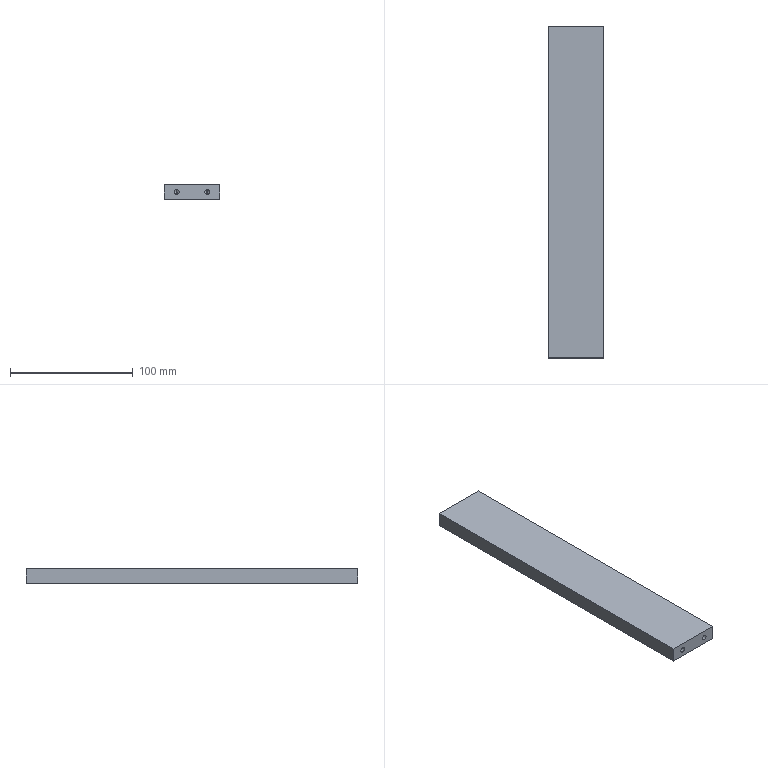Component | SolidWorks | PressingMechanism-01-1 | 1 solid | 22 faces | box 45 x 270 x 12 mm | volume 145001 mm3 | cylinder 8 | cone 8 | plane 6 | commonest cylinder face diameters 4.2 x8
build123d program:
from build123d import *

# Parameters (mm, degrees)
SKETCH1_W             = 45
SKETCH1_H             = 270
EXTRUDE1_DEPTH        = 6
M5_TAPPED_HOLE1_D     = 4.2
M5_TAPPED_HOLE1_DEPTH = 14
M5_TAPPED_HOLE1_TIP   = 1.262
M5_TAPPED_HOLE2_D     = 4.2
M5_TAPPED_HOLE2_DEPTH = 14
M5_TAPPED_HOLE2_TIP   = 1.262


with BuildPart() as part:
    # Sketch1 → Extrude1 (new, symmetric)
    with BuildSketch(Plane.XY):
        Rectangle(SKETCH1_W, SKETCH1_H)
    extrude(amount=EXTRUDE1_DEPTH, both=True)

    # M5 Tapped Hole1
    with Locations(Plane(origin=(0, 135, 0), x_dir=(1, 0, 0), z_dir=(0, 1, 0))):
        with Locations((-12.5, 0), (12.5, 0)):
            Hole(M5_TAPPED_HOLE1_D / 2, depth=M5_TAPPED_HOLE1_DEPTH)
            with Locations((0, 0, -(M5_TAPPED_HOLE1_DEPTH + M5_TAPPED_HOLE1_TIP / 2))):  # 118° drill point
                Cone(0, M5_TAPPED_HOLE1_D / 2, M5_TAPPED_HOLE1_TIP, mode=Mode.SUBTRACT)

    # M5 Tapped Hole2
    with Locations(Plane(origin=(0, -135, 0), x_dir=(-1, 0, 0), z_dir=(0, -1, 0))):
        with Locations((-12.5, 0), (12.5, 0)):
            Hole(M5_TAPPED_HOLE2_D / 2, depth=M5_TAPPED_HOLE2_DEPTH)
            with Locations((0, 0, -(M5_TAPPED_HOLE2_DEPTH + M5_TAPPED_HOLE2_TIP / 2))):  # 118° drill point
                Cone(0, M5_TAPPED_HOLE2_D / 2, M5_TAPPED_HOLE2_TIP, mode=Mode.SUBTRACT)


solid = part.part

# Placed as in the assembly
solid = solid.moved(Location((207.5, -90, 51), (0, 0, 0)))
STEP:
#1=CARTESIAN_POINT('',(8.661,1.22,1.925));
#2=VERTEX_POINT('',#1);
#3=CARTESIAN_POINT('',(8.661,1.22,2.091));
#4=VERTEX_POINT('',#3);
#5=CARTESIAN_POINT('',(8.661,1.22,2.008));
#6=DIRECTION('',(-0.,1.,-0.));
#7=DIRECTION('',(0.,0.,1.));
#8=AXIS2_PLACEMENT_3D('',#5,#6,#7);
#9=CIRCLE('',#8,0.08268);
#10=EDGE_CURVE('',#2,#4,#9,.T.);
#11=ORIENTED_EDGE('',*,*,#10,.F.);
#12=CARTESIAN_POINT('',(8.661,1.772,1.925));
#13=VERTEX_POINT('',#12);
#14=CARTESIAN_POINT('',(8.661,1.772,1.925));
#15=DIRECTION('',(-0.,1.,-0.));
#16=VECTOR('',#15,39.37);
#17=LINE('',#14,#16);
#18=EDGE_CURVE('',#2,#13,#17,.T.);
#19=ORIENTED_EDGE('',*,*,#18,.T.);
#20=CARTESIAN_POINT('',(8.661,1.772,2.091));
#21=VERTEX_POINT('',#20);
#22=CARTESIAN_POINT('',(8.661,1.772,2.008));
#23=DIRECTION('',(-0.,1.,-0.));
#24=DIRECTION('',(0.,0.,1.));
#25=AXIS2_PLACEMENT_3D('',#22,#23,#24);
#26=CIRCLE('',#25,0.08268);
#27=EDGE_CURVE('',#13,#21,#26,.T.);
#28=ORIENTED_EDGE('',*,*,#27,.T.);
#29=CARTESIAN_POINT('',(8.661,1.772,2.091));
#30=DIRECTION('',(-0.,1.,-0.));
#31=VECTOR('',#30,39.37);
#32=LINE('',#29,#31);
#33=EDGE_CURVE('',#4,#21,#32,.T.);
#34=ORIENTED_EDGE('',*,*,#33,.F.);
#35=EDGE_LOOP('',(#11,#19,#28,#34));
#36=FACE_OUTER_BOUND('',#35,.T.);
#37=CARTESIAN_POINT('',(8.661,1.772,2.008));
#38=DIRECTION('',(-0.,1.,-0.));
#39=DIRECTION('',(0.,0.,1.));
#40=AXIS2_PLACEMENT_3D('',#37,#38,#39);
#41=CYLINDRICAL_SURFACE('',#40,0.08268);
#42=ADVANCED_FACE('',(#36),#41,.F.);
#43=CARTESIAN_POINT('',(8.661,1.171,2.008));
#44=VERTEX_POINT('',#43);
#45=CARTESIAN_POINT('',(8.661,1.22,2.091));
#46=DIRECTION('',(-0.,0.515,0.8572));
#47=VECTOR('',#46,39.37);
#48=LINE('',#45,#47);
#49=EDGE_CURVE('',#44,#4,#48,.T.);
#50=ORIENTED_EDGE('',*,*,#49,.F.);
#51=CARTESIAN_POINT('',(8.661,1.22,1.925));
#52=DIRECTION('',(0.,0.515,-0.8572));
#53=VECTOR('',#52,39.37);
#54=LINE('',#51,#53);
#55=EDGE_CURVE('',#44,#2,#54,.T.);
#56=ORIENTED_EDGE('',*,*,#55,.T.);
#57=ORIENTED_EDGE('',*,*,#10,.T.);
#58=EDGE_LOOP('',(#50,#56,#57));
#59=FACE_OUTER_BOUND('',#58,.T.);
#60=CARTESIAN_POINT('',(8.661,1.22,2.008));
#61=DIRECTION('',(-0.,1.,-0.));
#62=DIRECTION('',(0.,0.,1.));
#63=AXIS2_PLACEMENT_3D('',#60,#61,#62);
#64=CONICAL_SURFACE('',#63,0.08268,1.03);
#65=ADVANCED_FACE('',(#59),#64,.F.);
#66=CARTESIAN_POINT('',(7.677,1.22,1.925));
#67=VERTEX_POINT('',#66);
#68=CARTESIAN_POINT('',(7.677,1.22,2.091));
#69=VERTEX_POINT('',#68);
#70=CARTESIAN_POINT('',(7.677,1.22,2.008));
#71=DIRECTION('',(-0.,1.,-0.));
#72=DIRECTION('',(0.,0.,1.));
#73=AXIS2_PLACEMENT_3D('',#70,#71,#72);
#74=CIRCLE('',#73,0.08268);
#75=EDGE_CURVE('',#67,#69,#74,.T.);
#76=ORIENTED_EDGE('',*,*,#75,.F.);
#77=CARTESIAN_POINT('',(7.677,1.772,1.925));
#78=VERTEX_POINT('',#77);
#79=CARTESIAN_POINT('',(7.677,1.772,1.925));
#80=DIRECTION('',(-0.,1.,-0.));
#81=VECTOR('',#80,39.37);
#82=LINE('',#79,#81);
#83=EDGE_CURVE('',#67,#78,#82,.T.);
#84=ORIENTED_EDGE('',*,*,#83,.T.);
#85=CARTESIAN_POINT('',(7.677,1.772,2.091));
#86=VERTEX_POINT('',#85);
#87=CARTESIAN_POINT('',(7.677,1.772,2.008));
#88=DIRECTION('',(-0.,1.,-0.));
#89=DIRECTION('',(0.,0.,1.));
#90=AXIS2_PLACEMENT_3D('',#87,#88,#89);
#91=CIRCLE('',#90,0.08268);
#92=EDGE_CURVE('',#78,#86,#91,.T.);
#93=ORIENTED_EDGE('',*,*,#92,.T.);
#94=CARTESIAN_POINT('',(7.677,1.772,2.091));
#95=DIRECTION('',(-0.,1.,-0.));
#96=VECTOR('',#95,39.37);
#97=LINE('',#94,#96);
#98=EDGE_CURVE('',#69,#86,#97,.T.);
#99=ORIENTED_EDGE('',*,*,#98,.F.);
#100=EDGE_LOOP('',(#76,#84,#93,#99));
#101=FACE_OUTER_BOUND('',#100,.T.);
#102=CARTESIAN_POINT('',(7.677,1.772,2.008));
#103=DIRECTION('',(-0.,1.,-0.));
#104=DIRECTION('',(0.,0.,1.));
#105=AXIS2_PLACEMENT_3D('',#102,#103,#104);
#106=CYLINDRICAL_SURFACE('',#105,0.08268);
#107=ADVANCED_FACE('',(#101),#106,.F.);
#108=CARTESIAN_POINT('',(7.677,1.171,2.008));
#109=VERTEX_POINT('',#108);
#110=CARTESIAN_POINT('',(7.677,1.22,2.091));
#111=DIRECTION('',(-0.,0.515,0.8572));
#112=VECTOR('',#111,39.37);
#113=LINE('',#110,#112);
#114=EDGE_CURVE('',#109,#69,#113,.T.);
#115=ORIENTED_EDGE('',*,*,#114,.F.);
#116=CARTESIAN_POINT('',(7.677,1.22,1.925));
#117=DIRECTION('',(0.,0.515,-0.8572));
#118=VECTOR('',#117,39.37);
#119=LINE('',#116,#118);
#120=EDGE_CURVE('',#109,#67,#119,.T.);
#121=ORIENTED_EDGE('',*,*,#120,.T.);
#122=ORIENTED_EDGE('',*,*,#75,.T.);
#123=EDGE_LOOP('',(#115,#121,#122));
#124=FACE_OUTER_BOUND('',#123,.T.);
#125=CARTESIAN_POINT('',(7.677,1.22,2.008));
#126=DIRECTION('',(-0.,1.,-0.));
#127=DIRECTION('',(0.,0.,1.));
#128=AXIS2_PLACEMENT_3D('',#125,#126,#127);
#129=CONICAL_SURFACE('',#128,0.08268,1.03);
#130=ADVANCED_FACE('',(#124),#129,.F.);
#131=CARTESIAN_POINT('',(7.677,-8.307,2.091));
#132=VERTEX_POINT('',#131);
#133=CARTESIAN_POINT('',(7.677,-8.307,1.925));
#134=VERTEX_POINT('',#133);
#135=CARTESIAN_POINT('',(7.677,-8.307,2.008));
#136=DIRECTION('',(0.,-1.,0.));
#137=DIRECTION('',(0.,0.,-1.));
#138=AXIS2_PLACEMENT_3D('',#135,#136,#137);
#139=CIRCLE('',#138,0.08268);
#140=EDGE_CURVE('',#132,#134,#139,.T.);
#141=ORIENTED_EDGE('',*,*,#140,.F.);
#142=CARTESIAN_POINT('',(7.677,-8.858,2.091));
#143=VERTEX_POINT('',#142);
#144=CARTESIAN_POINT('',(7.677,-8.858,2.091));
#145=DIRECTION('',(0.,-1.,0.));
#146=VECTOR('',#145,39.37);
#147=LINE('',#144,#146);
#148=EDGE_CURVE('',#132,#143,#147,.T.);
#149=ORIENTED_EDGE('',*,*,#148,.T.);
#150=CARTESIAN_POINT('',(7.677,-8.858,1.925));
#151=VERTEX_POINT('',#150);
#152=CARTESIAN_POINT('',(7.677,-8.858,2.008));
#153=DIRECTION('',(0.,-1.,0.));
#154=DIRECTION('',(0.,0.,-1.));
#155=AXIS2_PLACEMENT_3D('',#152,#153,#154);
#156=CIRCLE('',#155,0.08268);
#157=EDGE_CURVE('',#143,#151,#156,.T.);
#158=ORIENTED_EDGE('',*,*,#157,.T.);
#159=CARTESIAN_POINT('',(7.677,-8.858,1.925));
#160=DIRECTION('',(0.,-1.,0.));
#161=VECTOR('',#160,39.37);
#162=LINE('',#159,#161);
#163=EDGE_CURVE('',#134,#151,#162,.T.);
#164=ORIENTED_EDGE('',*,*,#163,.F.);
#165=EDGE_LOOP('',(#141,#149,#158,#164));
#166=FACE_OUTER_BOUND('',#165,.T.);
#167=CARTESIAN_POINT('',(7.677,-8.858,2.008));
#168=DIRECTION('',(0.,-1.,0.));
#169=DIRECTION('',(0.,0.,-1.));
#170=AXIS2_PLACEMENT_3D('',#167,#168,#169);
#171=CYLINDRICAL_SURFACE('',#170,0.08268);
#172=ADVANCED_FACE('',(#166),#171,.F.);
#173=CARTESIAN_POINT('',(7.677,-8.257,2.008));
#174=VERTEX_POINT('',#173);
#175=CARTESIAN_POINT('',(7.677,-8.307,1.925));
#176=DIRECTION('',(0.,-0.515,-0.8572));
#177=VECTOR('',#176,39.37);
#178=LINE('',#175,#177);
#179=EDGE_CURVE('',#174,#134,#178,.T.);
#180=ORIENTED_EDGE('',*,*,#179,.F.);
#181=CARTESIAN_POINT('',(7.677,-8.307,2.091));
#182=DIRECTION('',(0.,-0.515,0.8572));
#183=VECTOR('',#182,39.37);
#184=LINE('',#181,#183);
#185=EDGE_CURVE('',#174,#132,#184,.T.);
#186=ORIENTED_EDGE('',*,*,#185,.T.);
#187=ORIENTED_EDGE('',*,*,#140,.T.);
#188=EDGE_LOOP('',(#180,#186,#187));
#189=FACE_OUTER_BOUND('',#188,.T.);
#190=CARTESIAN_POINT('',(7.677,-8.307,2.008));
#191=DIRECTION('',(0.,-1.,0.));
#192=DIRECTION('',(0.,0.,-1.));
#193=AXIS2_PLACEMENT_3D('',#190,#191,#192);
#194=CONICAL_SURFACE('',#193,0.08268,1.03);
#195=ADVANCED_FACE('',(#189),#194,.F.);
#196=CARTESIAN_POINT('',(8.661,-8.307,2.091));
#197=VERTEX_POINT('',#196);
#198=CARTESIAN_POINT('',(8.661,-8.307,1.925));
#199=VERTEX_POINT('',#198);
#200=CARTESIAN_POINT('',(8.661,-8.307,2.008));
#201=DIRECTION('',(0.,-1.,0.));
#202=DIRECTION('',(0.,0.,-1.));
#203=AXIS2_PLACEMENT_3D('',#200,#201,#202);
#204=CIRCLE('',#203,0.08268);
#205=EDGE_CURVE('',#197,#199,#204,.T.);
#206=ORIENTED_EDGE('',*,*,#205,.F.);
#207=CARTESIAN_POINT('',(8.661,-8.858,2.091));
#208=VERTEX_POINT('',#207);
#209=CARTESIAN_POINT('',(8.661,-8.858,2.091));
#210=DIRECTION('',(0.,-1.,0.));
#211=VECTOR('',#210,39.37);
#212=LINE('',#209,#211);
#213=EDGE_CURVE('',#197,#208,#212,.T.);
#214=ORIENTED_EDGE('',*,*,#213,.T.);
#215=CARTESIAN_POINT('',(8.661,-8.858,1.925));
#216=VERTEX_POINT('',#215);
#217=CARTESIAN_POINT('',(8.661,-8.858,2.008));
#218=DIRECTION('',(0.,-1.,0.));
#219=DIRECTION('',(0.,0.,-1.));
#220=AXIS2_PLACEMENT_3D('',#217,#218,#219);
#221=CIRCLE('',#220,0.08268);
#222=EDGE_CURVE('',#208,#216,#221,.T.);
#223=ORIENTED_EDGE('',*,*,#222,.T.);
#224=CARTESIAN_POINT('',(8.661,-8.858,1.925));
#225=DIRECTION('',(0.,-1.,0.));
#226=VECTOR('',#225,39.37);
#227=LINE('',#224,#226);
#228=EDGE_CURVE('',#199,#216,#227,.T.);
#229=ORIENTED_EDGE('',*,*,#228,.F.);
#230=EDGE_LOOP('',(#206,#214,#223,#229));
#231=FACE_OUTER_BOUND('',#230,.T.);
#232=CARTESIAN_POINT('',(8.661,-8.858,2.008));
#233=DIRECTION('',(0.,-1.,0.));
#234=DIRECTION('',(0.,0.,-1.));
#235=AXIS2_PLACEMENT_3D('',#232,#233,#234);
#236=CYLINDRICAL_SURFACE('',#235,0.08268);
#237=ADVANCED_FACE('',(#231),#236,.F.);
#238=CARTESIAN_POINT('',(8.661,-8.257,2.008));
#239=VERTEX_POINT('',#238);
#240=CARTESIAN_POINT('',(8.661,-8.307,1.925));
#241=DIRECTION('',(0.,-0.515,-0.8572));
#242=VECTOR('',#241,39.37);
#243=LINE('',#240,#242);
#244=EDGE_CURVE('',#239,#199,#243,.T.);
#245=ORIENTED_EDGE('',*,*,#244,.F.);
#246=CARTESIAN_POINT('',(8.661,-8.307,2.091));
#247=DIRECTION('',(0.,-0.515,0.8572));
#248=VECTOR('',#247,39.37);
#249=LINE('',#246,#248);
#250=EDGE_CURVE('',#239,#197,#249,.T.);
#251=ORIENTED_EDGE('',*,*,#250,.T.);
#252=ORIENTED_EDGE('',*,*,#205,.T.);
#253=EDGE_LOOP('',(#245,#251,#252));
#254=FACE_OUTER_BOUND('',#253,.T.);
#255=CARTESIAN_POINT('',(8.661,-8.307,2.008));
#256=DIRECTION('',(0.,-1.,0.));
#257=DIRECTION('',(0.,0.,-1.));
#258=AXIS2_PLACEMENT_3D('',#255,#256,#257);
#259=CONICAL_SURFACE('',#258,0.08268,1.03);
#260=ADVANCED_FACE('',(#254),#259,.F.);
#261=CARTESIAN_POINT('',(7.283,-8.858,2.244));
#262=VERTEX_POINT('',#261);
#263=CARTESIAN_POINT('',(7.283,1.772,2.244));
#264=VERTEX_POINT('',#263);
#265=CARTESIAN_POINT('',(7.283,-8.858,2.244));
#266=DIRECTION('',(-0.,1.,-0.));
#267=VECTOR('',#266,39.37);
#268=LINE('',#265,#267);
#269=EDGE_CURVE('',#262,#264,#268,.T.);
#270=ORIENTED_EDGE('',*,*,#269,.T.);
#271=CARTESIAN_POINT('',(7.283,1.772,1.772));
#272=VERTEX_POINT('',#271);
#273=CARTESIAN_POINT('',(7.283,1.772,1.772));
#274=DIRECTION('',(-0.,0.,1.));
#275=VECTOR('',#274,39.37);
#276=LINE('',#273,#275);
#277=EDGE_CURVE('',#272,#264,#276,.T.);
#278=ORIENTED_EDGE('',*,*,#277,.F.);
#279=CARTESIAN_POINT('',(7.283,-8.858,1.772));
#280=VERTEX_POINT('',#279);
#281=CARTESIAN_POINT('',(7.283,-8.858,1.772));
#282=DIRECTION('',(-0.,1.,-0.));
#283=VECTOR('',#282,39.37);
#284=LINE('',#281,#283);
#285=EDGE_CURVE('',#280,#272,#284,.T.);
#286=ORIENTED_EDGE('',*,*,#285,.F.);
#287=CARTESIAN_POINT('',(7.283,-8.858,1.772));
#288=DIRECTION('',(-0.,0.,1.));
#289=VECTOR('',#288,39.37);
#290=LINE('',#287,#289);
#291=EDGE_CURVE('',#280,#262,#290,.T.);
#292=ORIENTED_EDGE('',*,*,#291,.T.);
#293=EDGE_LOOP('',(#270,#278,#286,#292));
#294=FACE_OUTER_BOUND('',#293,.T.);
#295=CARTESIAN_POINT('',(7.283,-8.858,1.772));
#296=DIRECTION('',(1.,0.,0.));
#297=DIRECTION('',(-0.,0.,1.));
#298=AXIS2_PLACEMENT_3D('',#295,#296,#297);
#299=PLANE('',#298);
#300=ADVANCED_FACE('',(#294),#299,.F.);
#301=CARTESIAN_POINT('',(8.661,1.772,2.008));
#302=DIRECTION('',(-0.,1.,-0.));
#303=DIRECTION('',(0.,0.,1.));
#304=AXIS2_PLACEMENT_3D('',#301,#302,#303);
#305=CIRCLE('',#304,0.08268);
#306=EDGE_CURVE('',#21,#13,#305,.T.);
#307=ORIENTED_EDGE('',*,*,#306,.F.);
#308=ORIENTED_EDGE('',*,*,#27,.F.);
#309=EDGE_LOOP('',(#307,#308));
#310=FACE_BOUND('',#309,.T.);
#311=CARTESIAN_POINT('',(7.677,1.772,2.008));
#312=DIRECTION('',(-0.,1.,-0.));
#313=DIRECTION('',(0.,0.,1.));
#314=AXIS2_PLACEMENT_3D('',#311,#312,#313);
#315=CIRCLE('',#314,0.08268);
#316=EDGE_CURVE('',#86,#78,#315,.T.);
#317=ORIENTED_EDGE('',*,*,#316,.F.);
#318=ORIENTED_EDGE('',*,*,#92,.F.);
#319=EDGE_LOOP('',(#317,#318));
#320=FACE_BOUND('',#319,.T.);
#321=CARTESIAN_POINT('',(9.055,1.772,2.244));
#322=VERTEX_POINT('',#321);
#323=CARTESIAN_POINT('',(7.283,1.772,2.244));
#324=DIRECTION('',(1.,0.,0.));
#325=VECTOR('',#324,39.37);
#326=LINE('',#323,#325);
#327=EDGE_CURVE('',#264,#322,#326,.T.);
#328=ORIENTED_EDGE('',*,*,#327,.T.);
#329=CARTESIAN_POINT('',(9.055,1.772,1.772));
#330=VERTEX_POINT('',#329);
#331=CARTESIAN_POINT('',(9.055,1.772,1.772));
#332=DIRECTION('',(-0.,0.,1.));
#333=VECTOR('',#332,39.37);
#334=LINE('',#331,#333);
#335=EDGE_CURVE('',#330,#322,#334,.T.);
#336=ORIENTED_EDGE('',*,*,#335,.F.);
#337=CARTESIAN_POINT('',(7.283,1.772,1.772));
#338=DIRECTION('',(1.,0.,0.));
#339=VECTOR('',#338,39.37);
#340=LINE('',#337,#339);
#341=EDGE_CURVE('',#272,#330,#340,.T.);
#342=ORIENTED_EDGE('',*,*,#341,.F.);
#343=ORIENTED_EDGE('',*,*,#277,.T.);
#344=EDGE_LOOP('',(#328,#336,#342,#343));
#345=FACE_OUTER_BOUND('',#344,.T.);
#346=CARTESIAN_POINT('',(7.283,1.772,1.772));
#347=DIRECTION('',(0.,-1.,0.));
#348=DIRECTION('',(0.,-0.,-1.));
#349=AXIS2_PLACEMENT_3D('',#346,#347,#348);
#350=PLANE('',#349);
#351=ADVANCED_FACE('',(#310,#320,#345),#350,.F.);
#352=CARTESIAN_POINT('',(9.055,-8.858,2.244));
#353=VERTEX_POINT('',#352);
#354=CARTESIAN_POINT('',(9.055,-8.858,2.244));
#355=DIRECTION('',(0.,-1.,0.));
#356=VECTOR('',#355,39.37);
#357=LINE('',#354,#356);
#358=EDGE_CURVE('',#322,#353,#357,.T.);
#359=ORIENTED_EDGE('',*,*,#358,.T.);
#360=CARTESIAN_POINT('',(9.055,-8.858,1.772));
#361=VERTEX_POINT('',#360);
#362=CARTESIAN_POINT('',(9.055,-8.858,1.772));
#363=DIRECTION('',(-0.,0.,1.));
#364=VECTOR('',#363,39.37);
#365=LINE('',#362,#364);
#366=EDGE_CURVE('',#361,#353,#365,.T.);
#367=ORIENTED_EDGE('',*,*,#366,.F.);
#368=CARTESIAN_POINT('',(9.055,-8.858,1.772));
#369=DIRECTION('',(0.,-1.,0.));
#370=VECTOR('',#369,39.37);
#371=LINE('',#368,#370);
#372=EDGE_CURVE('',#330,#361,#371,.T.);
#373=ORIENTED_EDGE('',*,*,#372,.F.);
#374=ORIENTED_EDGE('',*,*,#335,.T.);
#375=EDGE_LOOP('',(#359,#367,#373,#374));
#376=FACE_OUTER_BOUND('',#375,.T.);
#377=CARTESIAN_POINT('',(9.055,-8.858,1.772));
#378=DIRECTION('',(-1.,-0.,-0.));
#379=DIRECTION('',(0.,-0.,-1.));
#380=AXIS2_PLACEMENT_3D('',#377,#378,#379);
#381=PLANE('',#380);
#382=ADVANCED_FACE('',(#376),#381,.F.);
#383=CARTESIAN_POINT('',(7.677,-8.858,2.008));
#384=DIRECTION('',(0.,-1.,0.));
#385=DIRECTION('',(0.,0.,-1.));
#386=AXIS2_PLACEMENT_3D('',#383,#384,#385);
#387=CIRCLE('',#386,0.08268);
#388=EDGE_CURVE('',#151,#143,#387,.T.);
#389=ORIENTED_EDGE('',*,*,#388,.F.);
#390=ORIENTED_EDGE('',*,*,#157,.F.);
#391=EDGE_LOOP('',(#389,#390));
#392=FACE_BOUND('',#391,.T.);
#393=CARTESIAN_POINT('',(8.661,-8.858,2.008));
#394=DIRECTION('',(0.,-1.,0.));
#395=DIRECTION('',(0.,0.,-1.));
#396=AXIS2_PLACEMENT_3D('',#393,#394,#395);
#397=CIRCLE('',#396,0.08268);
#398=EDGE_CURVE('',#216,#208,#397,.T.);
#399=ORIENTED_EDGE('',*,*,#398,.F.);
#400=ORIENTED_EDGE('',*,*,#222,.F.);
#401=EDGE_LOOP('',(#399,#400));
#402=FACE_BOUND('',#401,.T.);
#403=CARTESIAN_POINT('',(7.283,-8.858,2.244));
#404=DIRECTION('',(-1.,-0.,-0.));
#405=VECTOR('',#404,39.37);
#406=LINE('',#403,#405);
#407=EDGE_CURVE('',#353,#262,#406,.T.);
#408=ORIENTED_EDGE('',*,*,#407,.T.);
#409=ORIENTED_EDGE('',*,*,#291,.F.);
#410=CARTESIAN_POINT('',(7.283,-8.858,1.772));
#411=DIRECTION('',(-1.,-0.,-0.));
#412=VECTOR('',#411,39.37);
#413=LINE('',#410,#412);
#414=EDGE_CURVE('',#361,#280,#413,.T.);
#415=ORIENTED_EDGE('',*,*,#414,.F.);
#416=ORIENTED_EDGE('',*,*,#366,.T.);
#417=EDGE_LOOP('',(#408,#409,#415,#416));
#418=FACE_OUTER_BOUND('',#417,.T.);
#419=CARTESIAN_POINT('',(7.283,-8.858,1.772));
#420=DIRECTION('',(-0.,1.,-0.));
#421=DIRECTION('',(-0.,0.,1.));
#422=AXIS2_PLACEMENT_3D('',#419,#420,#421);
#423=PLANE('',#422);
#424=ADVANCED_FACE('',(#392,#402,#418),#423,.F.);
#425=ORIENTED_EDGE('',*,*,#285,.T.);
#426=ORIENTED_EDGE('',*,*,#341,.T.);
#427=ORIENTED_EDGE('',*,*,#372,.T.);
#428=ORIENTED_EDGE('',*,*,#414,.T.);
#429=EDGE_LOOP('',(#425,#426,#427,#428));
#430=FACE_OUTER_BOUND('',#429,.T.);
#431=CARTESIAN_POINT('',(8.169,-3.543,1.772));
#432=DIRECTION('',(0.,-0.,-1.));
#433=DIRECTION('',(1.,0.,0.));
#434=AXIS2_PLACEMENT_3D('',#431,#432,#433);
#435=PLANE('',#434);
#436=ADVANCED_FACE('',(#430),#435,.T.);
#437=ORIENTED_EDGE('',*,*,#269,.F.);
#438=ORIENTED_EDGE('',*,*,#407,.F.);
#439=ORIENTED_EDGE('',*,*,#358,.F.);
#440=ORIENTED_EDGE('',*,*,#327,.F.);
#441=EDGE_LOOP('',(#437,#438,#439,#440));
#442=FACE_OUTER_BOUND('',#441,.T.);
#443=CARTESIAN_POINT('',(8.169,-3.543,2.244));
#444=DIRECTION('',(0.,-0.,-1.));
#445=DIRECTION('',(1.,0.,0.));
#446=AXIS2_PLACEMENT_3D('',#443,#444,#445);
#447=PLANE('',#446);
#448=ADVANCED_FACE('',(#442),#447,.F.);
#449=ORIENTED_EDGE('',*,*,#250,.F.);
#450=ORIENTED_EDGE('',*,*,#244,.T.);
#451=CARTESIAN_POINT('',(8.661,-8.307,2.008));
#452=DIRECTION('',(0.,-1.,0.));
#453=DIRECTION('',(0.,0.,-1.));
#454=AXIS2_PLACEMENT_3D('',#451,#452,#453);
#455=CIRCLE('',#454,0.08268);
#456=EDGE_CURVE('',#199,#197,#455,.T.);
#457=ORIENTED_EDGE('',*,*,#456,.T.);
#458=EDGE_LOOP('',(#449,#450,#457));
#459=FACE_OUTER_BOUND('',#458,.T.);
#460=CARTESIAN_POINT('',(8.661,-8.307,2.008));
#461=DIRECTION('',(0.,-1.,0.));
#462=DIRECTION('',(0.,0.,-1.));
#463=AXIS2_PLACEMENT_3D('',#460,#461,#462);
#464=CONICAL_SURFACE('',#463,0.08268,1.03);
#465=ADVANCED_FACE('',(#459),#464,.F.);
#466=ORIENTED_EDGE('',*,*,#213,.F.);
#467=ORIENTED_EDGE('',*,*,#456,.F.);
#468=ORIENTED_EDGE('',*,*,#228,.T.);
#469=ORIENTED_EDGE('',*,*,#398,.T.);
#470=EDGE_LOOP('',(#466,#467,#468,#469));
#471=FACE_OUTER_BOUND('',#470,.T.);
#472=CARTESIAN_POINT('',(8.661,-8.858,2.008));
#473=DIRECTION('',(0.,-1.,0.));
#474=DIRECTION('',(0.,0.,-1.));
#475=AXIS2_PLACEMENT_3D('',#472,#473,#474);
#476=CYLINDRICAL_SURFACE('',#475,0.08268);
#477=ADVANCED_FACE('',(#471),#476,.F.);
#478=ORIENTED_EDGE('',*,*,#185,.F.);
#479=ORIENTED_EDGE('',*,*,#179,.T.);
#480=CARTESIAN_POINT('',(7.677,-8.307,2.008));
#481=DIRECTION('',(0.,-1.,0.));
#482=DIRECTION('',(0.,0.,-1.));
#483=AXIS2_PLACEMENT_3D('',#480,#481,#482);
#484=CIRCLE('',#483,0.08268);
#485=EDGE_CURVE('',#134,#132,#484,.T.);
#486=ORIENTED_EDGE('',*,*,#485,.T.);
#487=EDGE_LOOP('',(#478,#479,#486));
#488=FACE_OUTER_BOUND('',#487,.T.);
#489=CARTESIAN_POINT('',(7.677,-8.307,2.008));
#490=DIRECTION('',(0.,-1.,0.));
#491=DIRECTION('',(0.,0.,-1.));
#492=AXIS2_PLACEMENT_3D('',#489,#490,#491);
#493=CONICAL_SURFACE('',#492,0.08268,1.03);
#494=ADVANCED_FACE('',(#488),#493,.F.);
#495=ORIENTED_EDGE('',*,*,#148,.F.);
#496=ORIENTED_EDGE('',*,*,#485,.F.);
#497=ORIENTED_EDGE('',*,*,#163,.T.);
#498=ORIENTED_EDGE('',*,*,#388,.T.);
#499=EDGE_LOOP('',(#495,#496,#497,#498));
#500=FACE_OUTER_BOUND('',#499,.T.);
#501=CARTESIAN_POINT('',(7.677,-8.858,2.008));
#502=DIRECTION('',(0.,-1.,0.));
#503=DIRECTION('',(0.,0.,-1.));
#504=AXIS2_PLACEMENT_3D('',#501,#502,#503);
#505=CYLINDRICAL_SURFACE('',#504,0.08268);
#506=ADVANCED_FACE('',(#500),#505,.F.);
#507=ORIENTED_EDGE('',*,*,#120,.F.);
#508=ORIENTED_EDGE('',*,*,#114,.T.);
#509=CARTESIAN_POINT('',(7.677,1.22,2.008));
#510=DIRECTION('',(-0.,1.,-0.));
#511=DIRECTION('',(0.,0.,1.));
#512=AXIS2_PLACEMENT_3D('',#509,#510,#511);
#513=CIRCLE('',#512,0.08268);
#514=EDGE_CURVE('',#69,#67,#513,.T.);
#515=ORIENTED_EDGE('',*,*,#514,.T.);
#516=EDGE_LOOP('',(#507,#508,#515));
#517=FACE_OUTER_BOUND('',#516,.T.);
#518=CARTESIAN_POINT('',(7.677,1.22,2.008));
#519=DIRECTION('',(-0.,1.,-0.));
#520=DIRECTION('',(0.,0.,1.));
#521=AXIS2_PLACEMENT_3D('',#518,#519,#520);
#522=CONICAL_SURFACE('',#521,0.08268,1.03);
#523=ADVANCED_FACE('',(#517),#522,.F.);
#524=ORIENTED_EDGE('',*,*,#83,.F.);
#525=ORIENTED_EDGE('',*,*,#514,.F.);
#526=ORIENTED_EDGE('',*,*,#98,.T.);
#527=ORIENTED_EDGE('',*,*,#316,.T.);
#528=EDGE_LOOP('',(#524,#525,#526,#527));
#529=FACE_OUTER_BOUND('',#528,.T.);
#530=CARTESIAN_POINT('',(7.677,1.772,2.008));
#531=DIRECTION('',(-0.,1.,-0.));
#532=DIRECTION('',(0.,0.,1.));
#533=AXIS2_PLACEMENT_3D('',#530,#531,#532);
#534=CYLINDRICAL_SURFACE('',#533,0.08268);
#535=ADVANCED_FACE('',(#529),#534,.F.);
#536=ORIENTED_EDGE('',*,*,#55,.F.);
#537=ORIENTED_EDGE('',*,*,#49,.T.);
#538=CARTESIAN_POINT('',(8.661,1.22,2.008));
#539=DIRECTION('',(-0.,1.,-0.));
#540=DIRECTION('',(0.,0.,1.));
#541=AXIS2_PLACEMENT_3D('',#538,#539,#540);
#542=CIRCLE('',#541,0.08268);
#543=EDGE_CURVE('',#4,#2,#542,.T.);
#544=ORIENTED_EDGE('',*,*,#543,.T.);
#545=EDGE_LOOP('',(#536,#537,#544));
#546=FACE_OUTER_BOUND('',#545,.T.);
#547=CARTESIAN_POINT('',(8.661,1.22,2.008));
#548=DIRECTION('',(-0.,1.,-0.));
#549=DIRECTION('',(0.,0.,1.));
#550=AXIS2_PLACEMENT_3D('',#547,#548,#549);
#551=CONICAL_SURFACE('',#550,0.08268,1.03);
#552=ADVANCED_FACE('',(#546),#551,.F.);
#553=ORIENTED_EDGE('',*,*,#18,.F.);
#554=ORIENTED_EDGE('',*,*,#543,.F.);
#555=ORIENTED_EDGE('',*,*,#33,.T.);
#556=ORIENTED_EDGE('',*,*,#306,.T.);
#557=EDGE_LOOP('',(#553,#554,#555,#556));
#558=FACE_OUTER_BOUND('',#557,.T.);
#559=CARTESIAN_POINT('',(8.661,1.772,2.008));
#560=DIRECTION('',(-0.,1.,-0.));
#561=DIRECTION('',(0.,0.,1.));
#562=AXIS2_PLACEMENT_3D('',#559,#560,#561);
#563=CYLINDRICAL_SURFACE('',#562,0.08268);
#564=ADVANCED_FACE('',(#558),#563,.F.);
#565=CLOSED_SHELL('',(#42,#65,#107,#130,#172,#195,#237,#260,#300,#351,#382,#424,#436,#448,#465,#477,#494,#506,#523,#535,#552,#564));
#566=MANIFOLD_SOLID_BREP('',#565);
#567=CARTESIAN_POINT('',(0.,0.,0.));
#568=DIRECTION('',(0.,0.,1.));
#569=DIRECTION('',(1.,0.,0.));
#570=AXIS2_PLACEMENT_3D('',#567,#568,#569);
#571=(LENGTH_UNIT()NAMED_UNIT(*)SI_UNIT($,.METRE.));
#572=LENGTH_MEASURE_WITH_UNIT(LENGTH_MEASURE(0.0254),#571);
#573=DIMENSIONAL_EXPONENTS(1.,0.,0.,0.,0.,0.,0.);
#574=(CONVERSION_BASED_UNIT('',#572)LENGTH_UNIT()NAMED_UNIT(#573));
#575=UNCERTAINTY_MEASURE_WITH_UNIT(LENGTH_MEASURE(0.00001),#574,'','');
#576=(NAMED_UNIT(*)PLANE_ANGLE_UNIT()SI_UNIT($,.RADIAN.));
#577=(NAMED_UNIT(*)SI_UNIT($,.STERADIAN.)SOLID_ANGLE_UNIT());
#578=(GEOMETRIC_REPRESENTATION_CONTEXT(3)GLOBAL_UNCERTAINTY_ASSIGNED_CONTEXT((#575))GLOBAL_UNIT_ASSIGNED_CONTEXT((#574,#576,#577))REPRESENTATION_CONTEXT('',''));
#579=ADVANCED_BREP_SHAPE_REPRESENTATION('',(#566,#570),#578);
#580=COLOUR_RGB('',0.7922,0.8196,0.9333);
#581=FILL_AREA_STYLE_COLOUR('',#580);
#582=FILL_AREA_STYLE('',(#581));
#583=SURFACE_STYLE_FILL_AREA(#582);
#584=SURFACE_SIDE_STYLE('',(#583));
#585=SURFACE_STYLE_USAGE(.BOTH.,#584);
#586=PRESENTATION_STYLE_ASSIGNMENT((#585));
#587=STYLED_ITEM('',(#586),#566);
#588=PRESENTATION_LAYER_ASSIGNMENT('','',(#587));
#589=(LENGTH_UNIT()NAMED_UNIT(*)SI_UNIT($,.METRE.));
#590=LENGTH_MEASURE_WITH_UNIT(LENGTH_MEASURE(0.0254),#589);
#591=DIMENSIONAL_EXPONENTS(1.,0.,0.,0.,0.,0.,0.);
#592=(CONVERSION_BASED_UNIT('',#590)LENGTH_UNIT()NAMED_UNIT(#591));
#593=UNCERTAINTY_MEASURE_WITH_UNIT(LENGTH_MEASURE(0.00001),#592,'','');
#594=(NAMED_UNIT(*)PLANE_ANGLE_UNIT()SI_UNIT($,.RADIAN.));
#595=(NAMED_UNIT(*)SI_UNIT($,.STERADIAN.)SOLID_ANGLE_UNIT());
#596=(GEOMETRIC_REPRESENTATION_CONTEXT(3)GLOBAL_UNCERTAINTY_ASSIGNED_CONTEXT((#593))GLOBAL_UNIT_ASSIGNED_CONTEXT((#592,#594,#595))REPRESENTATION_CONTEXT('',''));
#597=MECHANICAL_DESIGN_GEOMETRIC_PRESENTATION_REPRESENTATION('',(#587),#596);